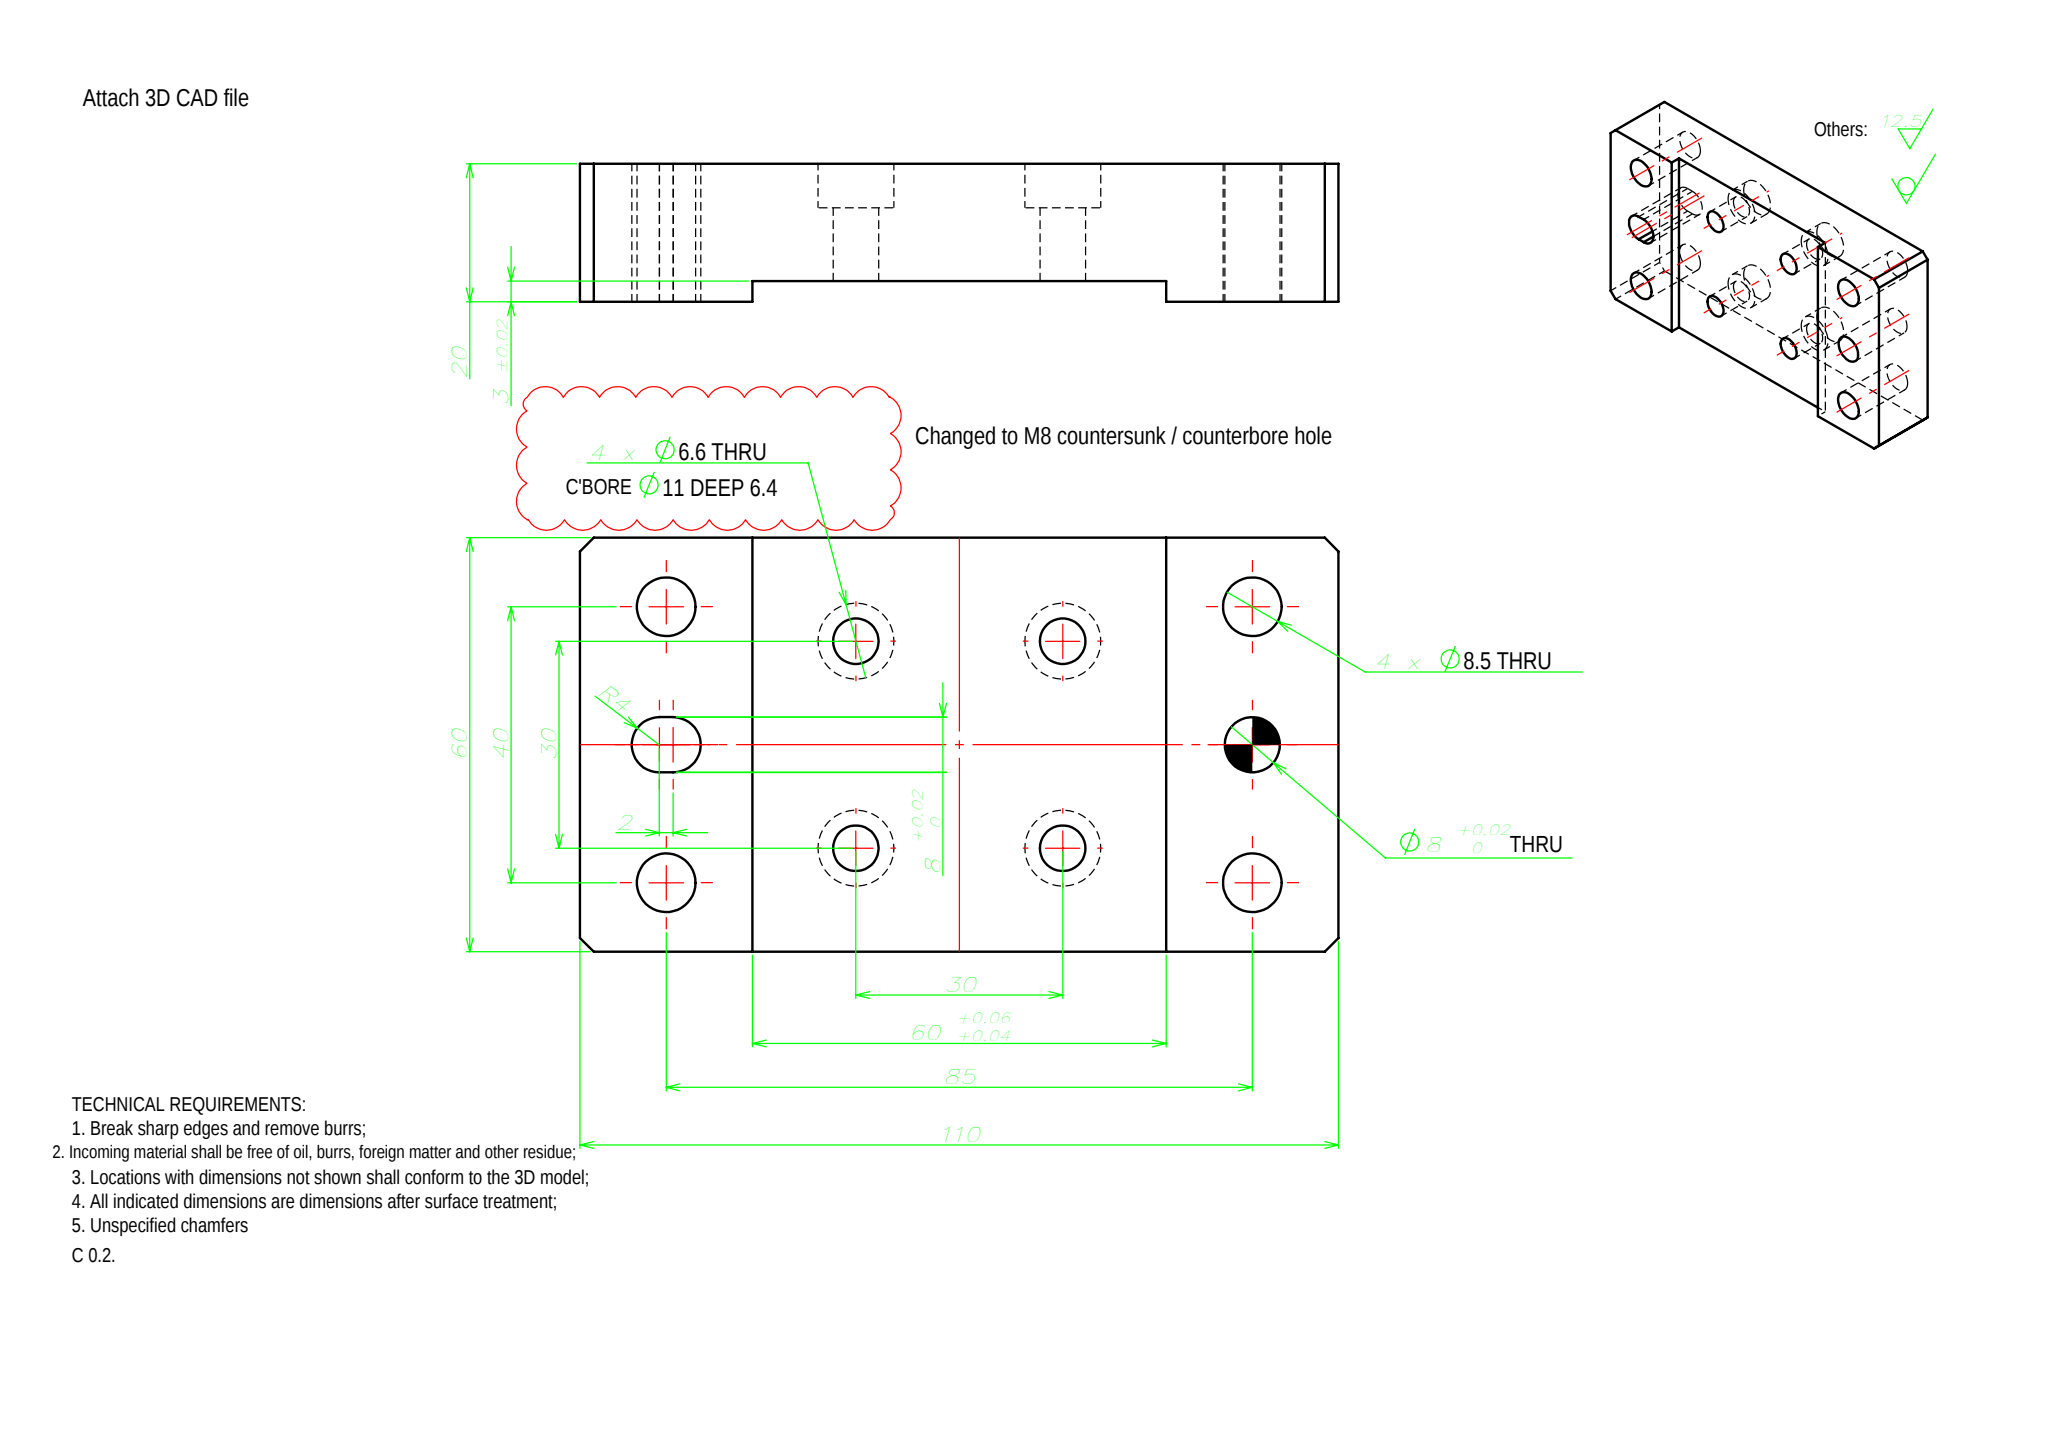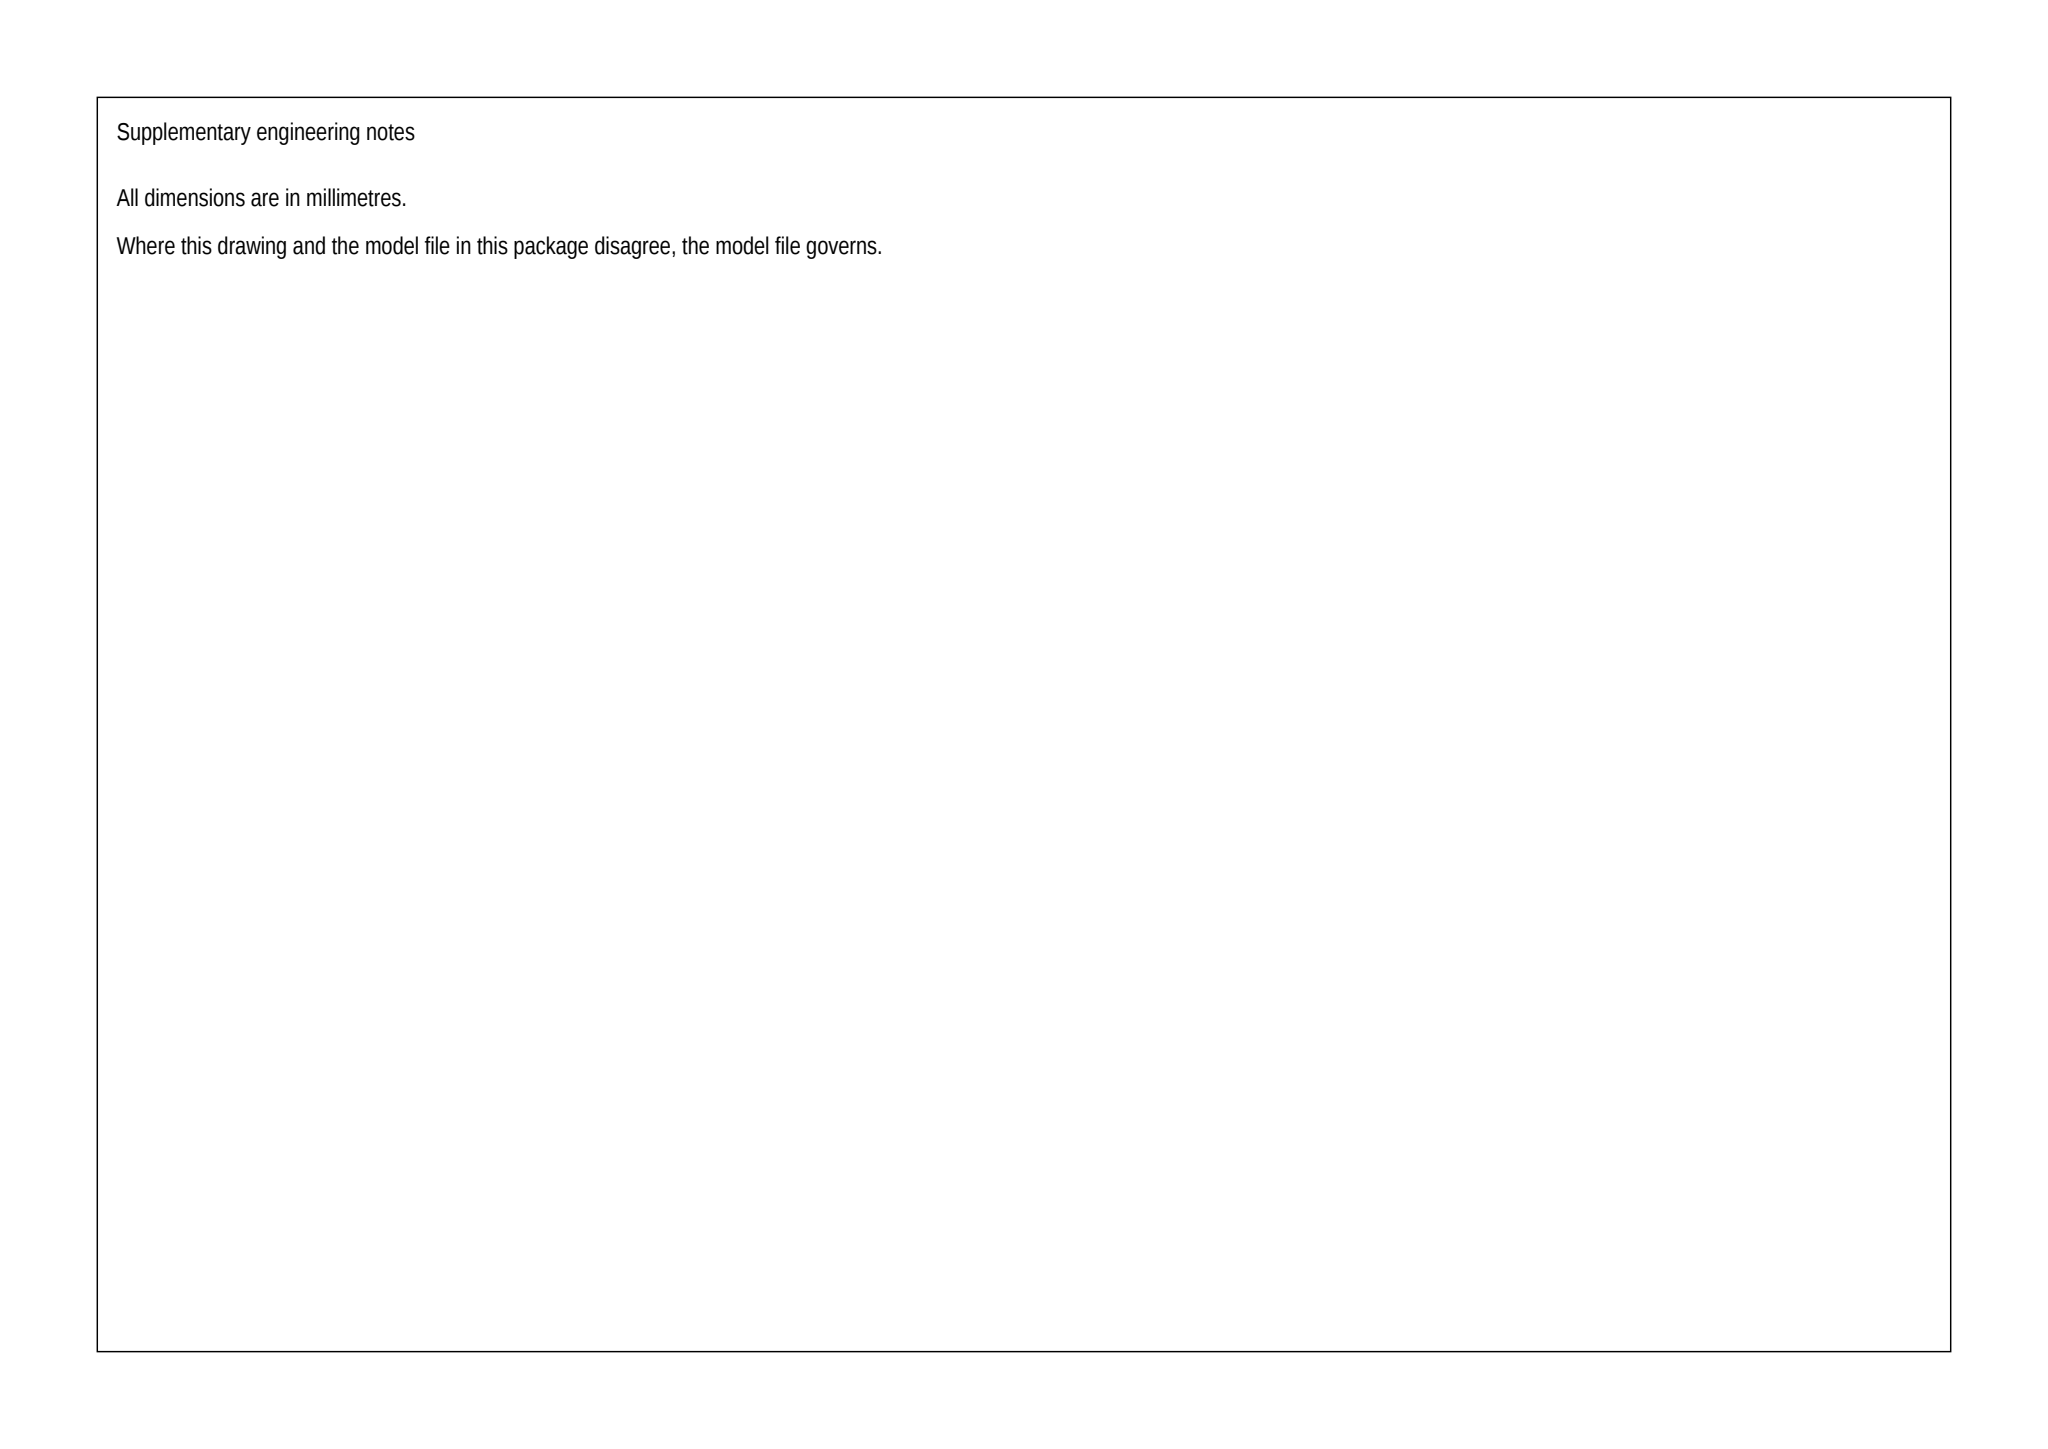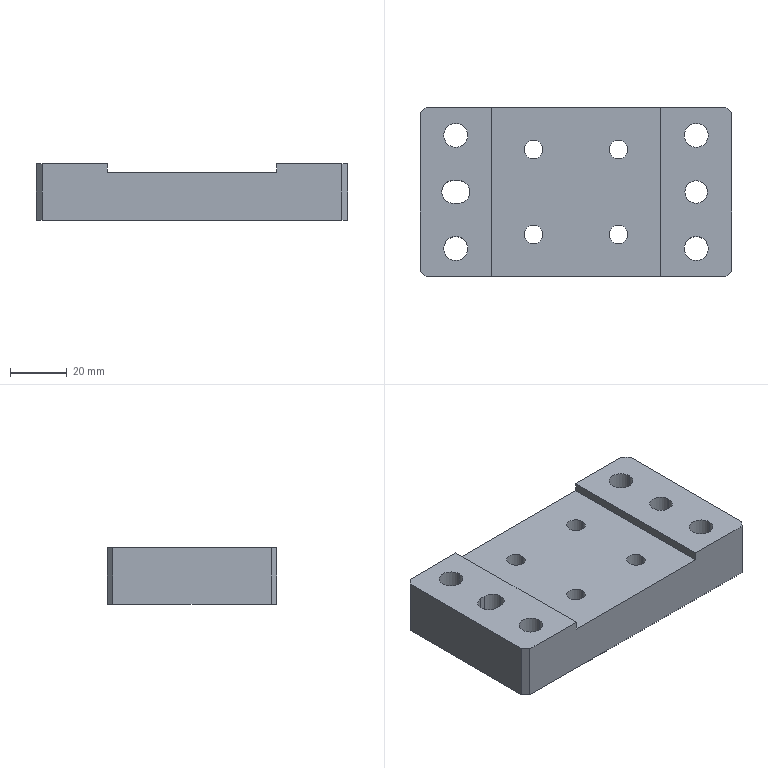Part | SolidWorks | mm | 1 solid | 49 faces | box 110 x 60 x 20 mm | volume 110286 mm3 | cylinder 29 | plane 20 | commonest cylinder face diameters 11 x8 6.6 x8 8.5 x8 8 x5
Drawing notes:
END PADS 25 WIDE EA END x 20 THK; CTR STEP 60 LG, FLOOR 17 FROM BOTTOM | from the solid: x-planes 0/25/85/110; z-planes 20 (ends) and 17 (middle); bbox 110x60x20
4X Ø6.6 THRU, CBORE Ø11 DP 6.4 FROM STEP FACE (17) | from the solid: Ø6.6 z L=10.6 + Ø11 z L=6.4 at (40,15),(40,45),(70,15),(70,45); 6.4+10.6=17
4X Ø8.5 THRU: CL 12.5 FROM EA END, 10 FROM EA SIDE | from the solid: Ø8.5 z THRU at (12.5,10),(12.5,50),(97.5,10),(97.5,50); bbox 110x60
Ø8 SLOT LH: CL 12.5 FROM LH END, 2 LG BTWN R4 ENDS; RH Ø8 CL 12.5 FROM RH END | from the solid: Ø8 z L=20 at x=11.5 & 13.5 (CL 12.5) and x=97.5, all y=30
4X Ø6.6 THRU, CBORE Ø11 DP 6.4; NO CSK - CLOUD CSK NOTE VOID | from the solid: Ø6.6 z-cyl L10.6 + Ø11 z-cyl L6.4 at (40,15)(40,45)(70,15)(70,45); cones[] empty
CBORE Ø11 DP 6.4 ENTERS FACE Z0 (OPP 17 STEP FACE), Ø6.6 THRU TO 17 | from the solid: Ø11 L6.4 spans z0-6.4 (z-plane 6.4 x4), Ø6.6 L10.6 spans 6.4-17.0; z-plane 17.0
4X Ø6.6 / CBORE Ø11 HOLES PLAIN - NO THREAD PER MODEL | from the solid: Only cylinders Ø6.6, Ø8, Ø8.5, Ø11; no helical/thread geometry in STEP
HOLE GRID: X 40 & 70 FROM LH EDGE, Y ±15 FROM 60 CL | from the solid: Ø6.6/Ø11 axes at x=40,70; y=15,45 of 60 width (CL y=30); bbox 110x60x20
build123d program:
from build123d import *

# Parameters (mm, degrees)
SKETCH1_W                                       = 110
SKETCH1_H                                       = 60
BOSS_EXTRUDE1_DEPTH                             = 20
SKETCH2_W                                       = 60
SKETCH2_H                                       = 19.774
CUT_EXTRUDE1_DEPTH                              = 60
CHAMFER1_SIZE                                   = 2
F_8_5_8_5_DIAMETER_HOLE1_D                      = 8.5
SKETCH8_R                                       = 4
CUT_EXTRUDE2_DEPTH                              = 71
M6_HEX_SOCKET_HEAD_CAP_SCREW_CBORE1_D           = 6.6
M6_HEX_SOCKET_HEAD_CAP_SCREW_CBORE1_CBORE_D     = 11
M6_HEX_SOCKET_HEAD_CAP_SCREW_CBORE1_CBORE_DEPTH = 6.4


with BuildPart() as part:
    # Sketch1 → Boss-Extrude1 (new body)
    with BuildSketch(Plane.XY):
        Rectangle(SKETCH1_W, SKETCH1_H)
    extrude(amount=BOSS_EXTRUDE1_DEPTH)

    # Sketch2 → Cut-Extrude1 (cut)
    with BuildSketch(Plane(origin=(0, 30, 0), x_dir=(1, 0, 0), z_dir=(0, 1, 0))):
        with Locations((0, -26.887)):
            Rectangle(SKETCH2_W, SKETCH2_H)
    extrude(amount=-CUT_EXTRUDE1_DEPTH, mode=Mode.SUBTRACT)

    # Chamfer1
    chamfer1_edges = [part.edges().sort_by_distance(p)[0] for p in [
        (55, -30, 10),
        (-55, -30, 10),
        (-55, 30, 10),
        (55, 30, 10),
    ]]
    chamfer(chamfer1_edges, length=CHAMFER1_SIZE)

    # 8.5 _8.5_ Diameter Hole1 (through all)
    with Locations(Plane.XY.offset(20)):
        with Locations((42.5, -20), (42.5, 20), (-42.5, 20), (-42.5, -20)):
            Hole(F_8_5_8_5_DIAMETER_HOLE1_D / 2)

    # Sketch8 → Cut-Extrude2 (cut)
    with BuildSketch(Plane.XY.offset(20)):
        with Locations((42.5, 0)):
            Circle(SKETCH8_R)
        with BuildLine():
            Line((-41.5, -4), (-43.5, -4))
            ThreePointArc((-43.5, -4), (-47.5, 0), (-43.5, 4))
            Line((-43.5, 4), (-41.5, 4))
            ThreePointArc((-41.5, 4), (-37.5, 0), (-41.5, -4))
        make_face()
    extrude(amount=-CUT_EXTRUDE2_DEPTH, mode=Mode.SUBTRACT)

    # M6 Hex Socket Head Cap Screw CBORE1 (through all)
    with Locations(Plane(origin=(0, 0, 0), x_dir=(-1, 0, 0), z_dir=(0, 0, -1))):
        with Locations((-15, 15), (15, 15), (15, -15), (-15, -15)):
            CounterBoreHole(M6_HEX_SOCKET_HEAD_CAP_SCREW_CBORE1_D / 2, M6_HEX_SOCKET_HEAD_CAP_SCREW_CBORE1_CBORE_D / 2, M6_HEX_SOCKET_HEAD_CAP_SCREW_CBORE1_CBORE_DEPTH)


solid = part.part